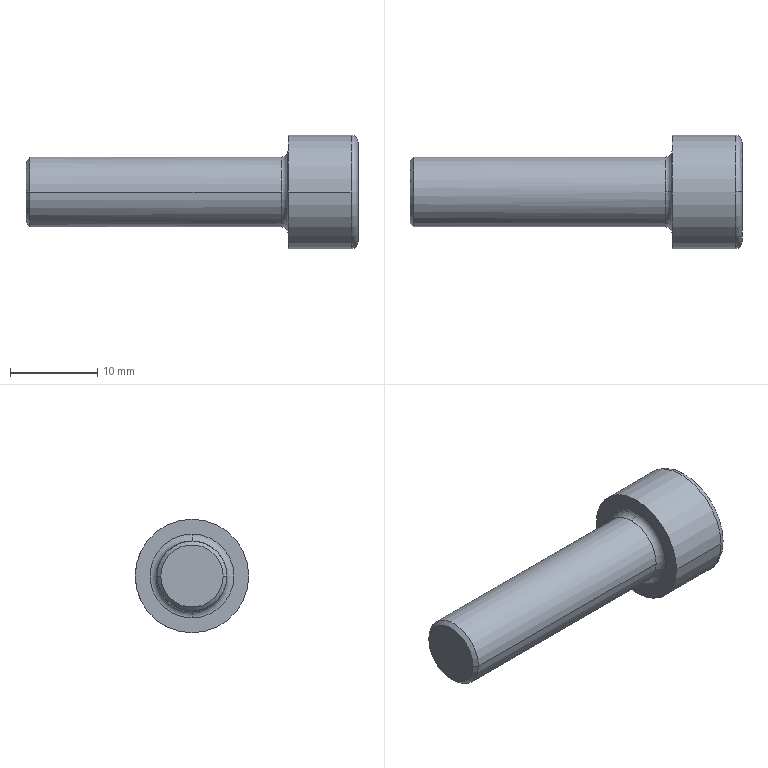Component | NX | M8X30 | 1 solid | 21 faces | volume 2416 mm3 | plane 9 | cylinder 4 | torus 4 | cone 4 | commonest cylinder face diameters 13 x2 8 x2